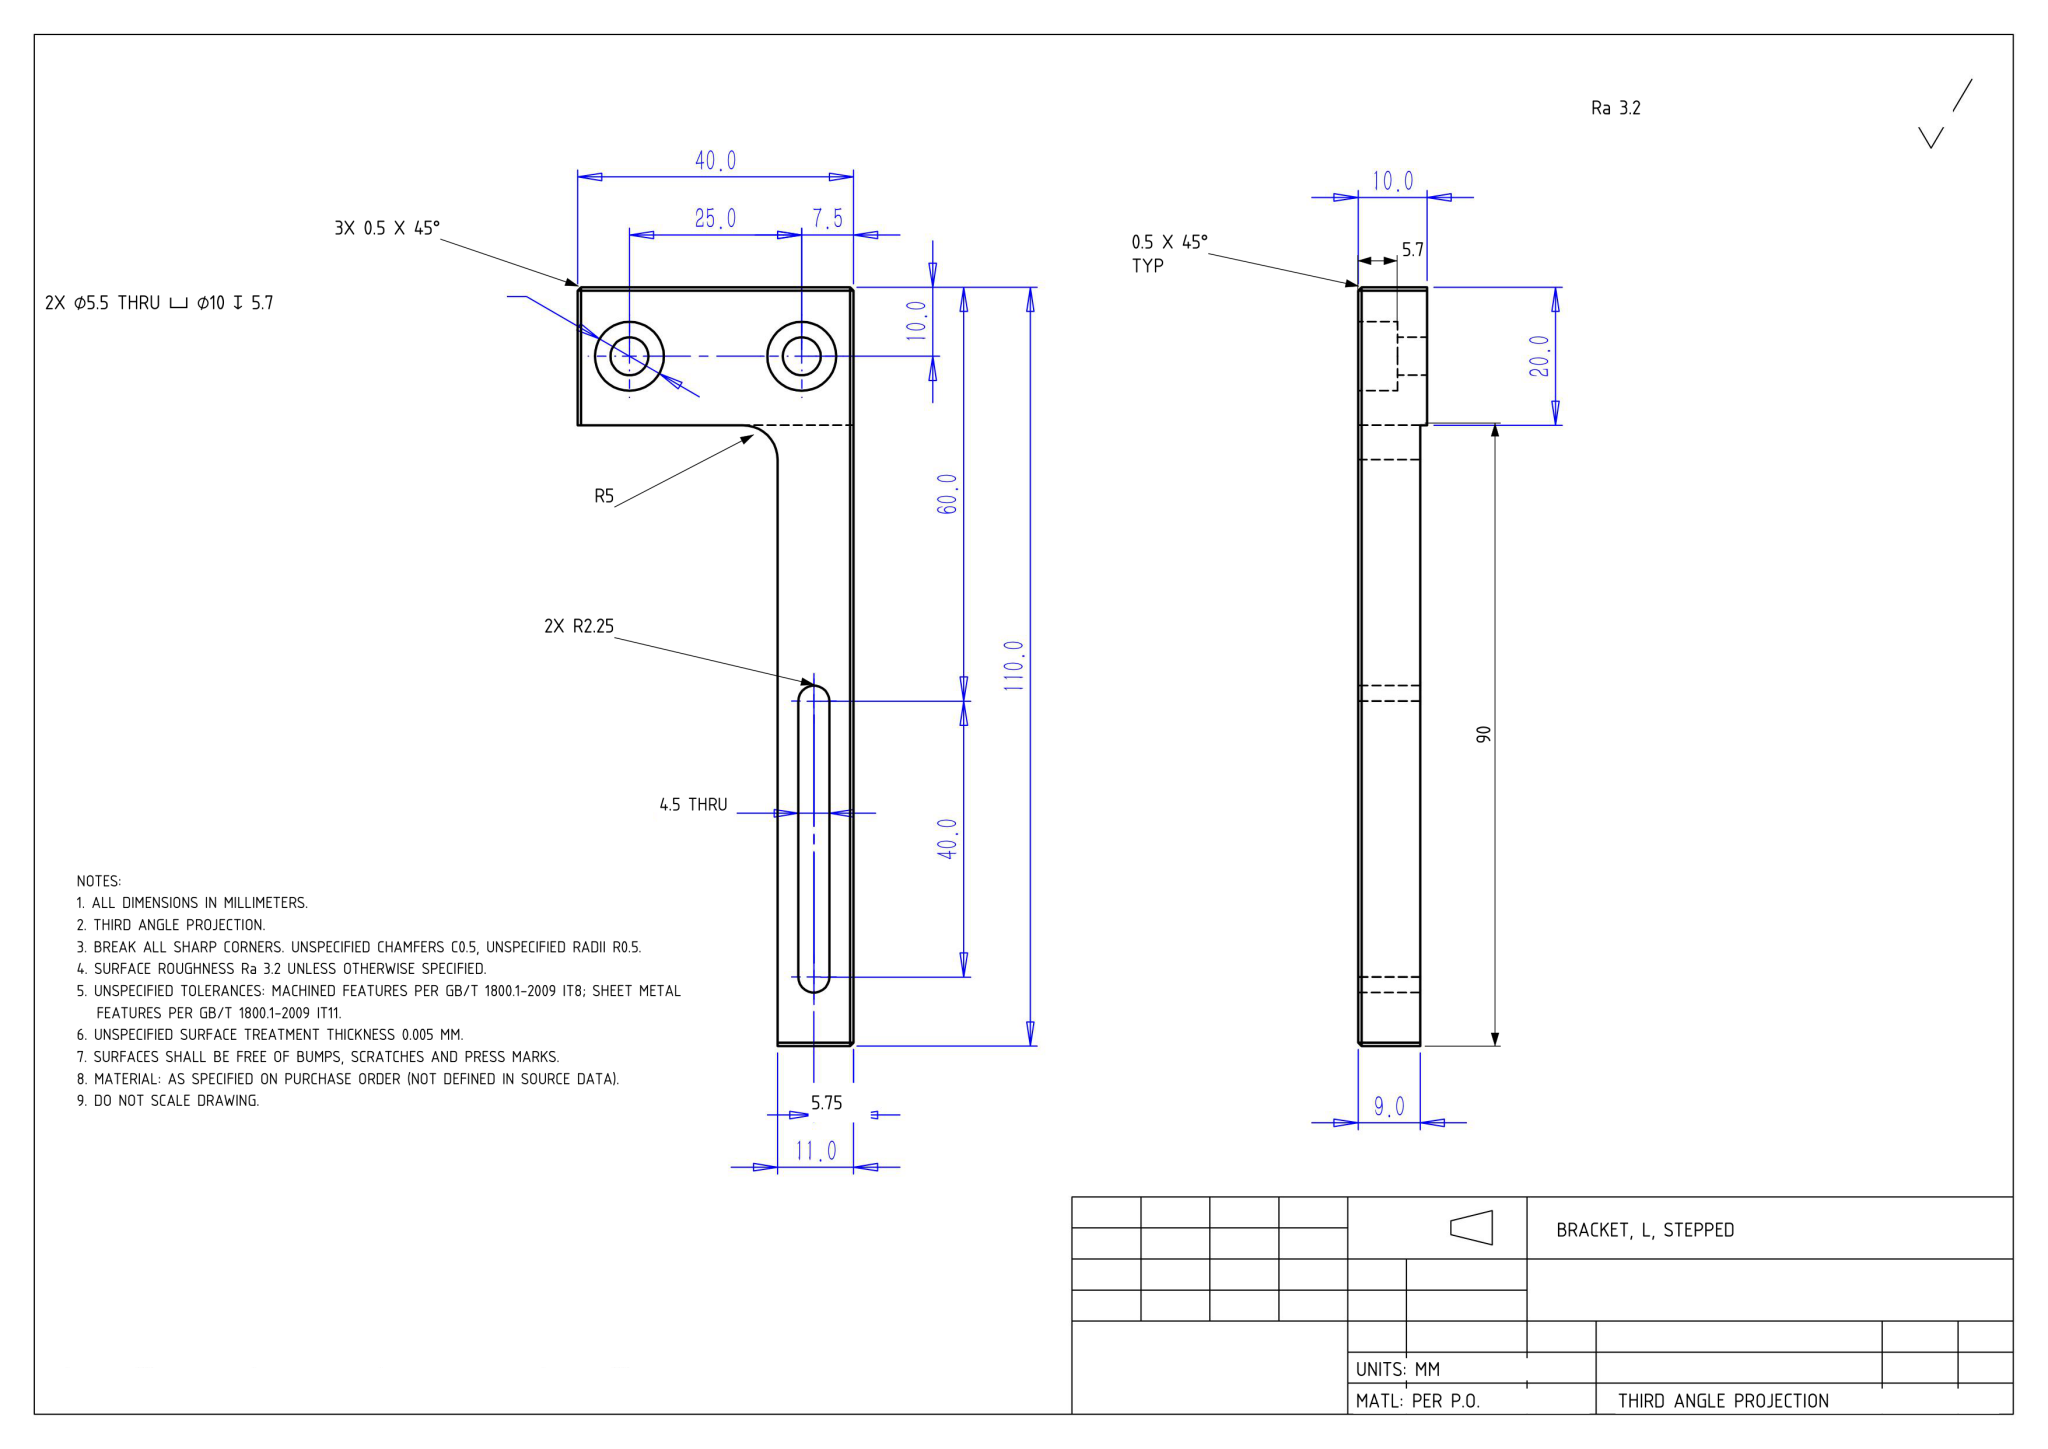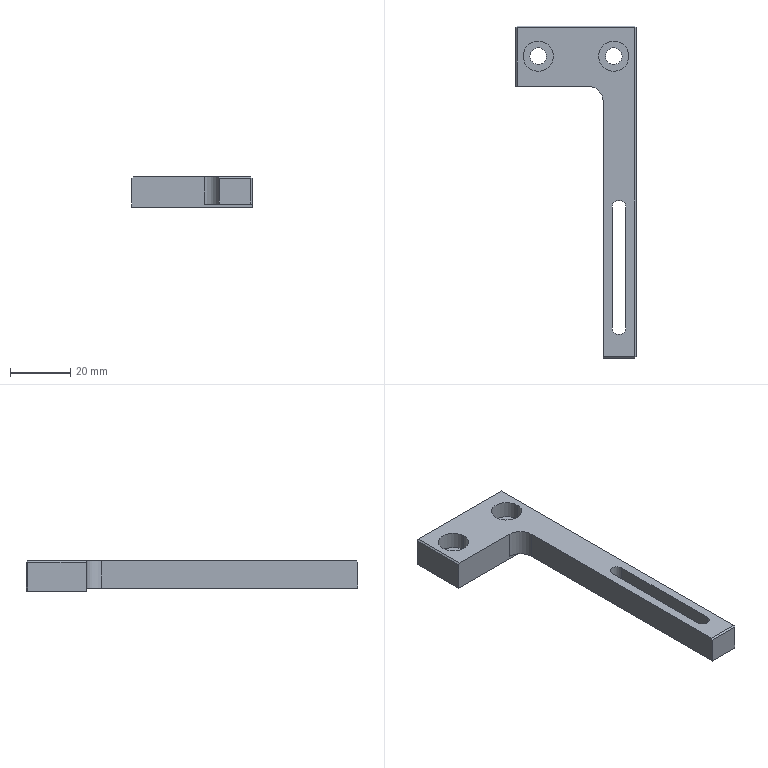Part | NX | mm | 1 solid | 34 faces | box 40 x 110 x 10 mm | volume 14069 mm3 | plane 23 | cylinder 11 | commonest cylinder face diameters 10 x5 5.5 x4 4.5 x2
STEP:
#1=COLOUR_RGB('',0.502,1.,1.);
#2=FILL_AREA_STYLE_COLOUR('',#1);
#3=FILL_AREA_STYLE('',(#2));
#4=SURFACE_STYLE_FILL_AREA(#3);
#5=SURFACE_SIDE_STYLE('',(#4));
#6=SURFACE_STYLE_USAGE(.BOTH.,#5);
#7=PRESENTATION_STYLE_ASSIGNMENT((#6));
#8=CARTESIAN_POINT('',(-17.5,45.,-0.7));
#9=VERTEX_POINT('',#8);
#10=CARTESIAN_POINT('',(-7.5,45.,-0.7));
#11=VERTEX_POINT('',#10);
#12=CARTESIAN_POINT('',(-12.5,45.,-0.7));
#13=DIRECTION('',(0.,0.,1.));
#14=DIRECTION('',(1.,0.,0.));
#15=AXIS2_PLACEMENT_3D('',#12,#13,#14);
#16=CIRCLE('',#15,5.);
#17=EDGE_CURVE('',#9,#11,#16,.T.);
#18=ORIENTED_EDGE('',*,*,#17,.F.);
#19=CARTESIAN_POINT('',(-17.5,45.,5.));
#20=VERTEX_POINT('',#19);
#21=CARTESIAN_POINT('',(-17.5,45.,5.));
#22=DIRECTION('',(0.,0.,1.));
#23=VECTOR('',#22,1000.);
#24=LINE('',#21,#23);
#25=EDGE_CURVE('',#9,#20,#24,.T.);
#26=ORIENTED_EDGE('',*,*,#25,.T.);
#27=CARTESIAN_POINT('',(-7.5,45.,5.));
#28=VERTEX_POINT('',#27);
#29=CARTESIAN_POINT('',(-12.5,45.,5.));
#30=DIRECTION('',(0.,0.,1.));
#31=DIRECTION('',(1.,0.,0.));
#32=AXIS2_PLACEMENT_3D('',#29,#30,#31);
#33=CIRCLE('',#32,5.);
#34=EDGE_CURVE('',#20,#28,#33,.T.);
#35=ORIENTED_EDGE('',*,*,#34,.T.);
#36=CARTESIAN_POINT('',(-7.5,45.,5.));
#37=DIRECTION('',(0.,0.,1.));
#38=VECTOR('',#37,1000.);
#39=LINE('',#36,#38);
#40=EDGE_CURVE('',#11,#28,#39,.T.);
#41=ORIENTED_EDGE('',*,*,#40,.F.);
#42=EDGE_LOOP('',(#18,#26,#35,#41));
#43=FACE_OUTER_BOUND('',#42,.T.);
#44=CARTESIAN_POINT('',(-12.5,45.,5.));
#45=DIRECTION('',(0.,0.,1.));
#46=DIRECTION('',(1.,0.,0.));
#47=AXIS2_PLACEMENT_3D('',#44,#45,#46);
#48=CYLINDRICAL_SURFACE('',#47,5.);
#49=ADVANCED_FACE('',(#43),#48,.F.);
#50=CARTESIAN_POINT('',(-15.25,45.,-5.));
#51=VERTEX_POINT('',#50);
#52=CARTESIAN_POINT('',(-9.75,45.,-5.));
#53=VERTEX_POINT('',#52);
#54=CARTESIAN_POINT('',(-12.5,45.,-5.));
#55=DIRECTION('',(0.,0.,1.));
#56=DIRECTION('',(1.,0.,0.));
#57=AXIS2_PLACEMENT_3D('',#54,#55,#56);
#58=CIRCLE('',#57,2.75);
#59=EDGE_CURVE('',#51,#53,#58,.T.);
#60=ORIENTED_EDGE('',*,*,#59,.F.);
#61=CARTESIAN_POINT('',(-15.25,45.,-0.7));
#62=VERTEX_POINT('',#61);
#63=CARTESIAN_POINT('',(-15.25,45.,5.));
#64=DIRECTION('',(0.,0.,1.));
#65=VECTOR('',#64,1000.);
#66=LINE('',#63,#65);
#67=EDGE_CURVE('',#51,#62,#66,.T.);
#68=ORIENTED_EDGE('',*,*,#67,.T.);
#69=CARTESIAN_POINT('',(-9.75,45.,-0.7));
#70=VERTEX_POINT('',#69);
#71=CARTESIAN_POINT('',(-12.5,45.,-0.7));
#72=DIRECTION('',(0.,0.,1.));
#73=DIRECTION('',(1.,0.,0.));
#74=AXIS2_PLACEMENT_3D('',#71,#72,#73);
#75=CIRCLE('',#74,2.75);
#76=EDGE_CURVE('',#62,#70,#75,.T.);
#77=ORIENTED_EDGE('',*,*,#76,.T.);
#78=CARTESIAN_POINT('',(-9.75,45.,5.));
#79=DIRECTION('',(0.,0.,1.));
#80=VECTOR('',#79,1000.);
#81=LINE('',#78,#80);
#82=EDGE_CURVE('',#53,#70,#81,.T.);
#83=ORIENTED_EDGE('',*,*,#82,.F.);
#84=EDGE_LOOP('',(#60,#68,#77,#83));
#85=FACE_OUTER_BOUND('',#84,.T.);
#86=CARTESIAN_POINT('',(-12.5,45.,5.));
#87=DIRECTION('',(0.,0.,1.));
#88=DIRECTION('',(1.,0.,0.));
#89=AXIS2_PLACEMENT_3D('',#86,#87,#88);
#90=CYLINDRICAL_SURFACE('',#89,2.75);
#91=ADVANCED_FACE('',(#85),#90,.F.);
#92=CARTESIAN_POINT('',(7.5,45.,-0.7));
#93=VERTEX_POINT('',#92);
#94=CARTESIAN_POINT('',(17.5,45.,-0.7));
#95=VERTEX_POINT('',#94);
#96=CARTESIAN_POINT('',(12.5,45.,-0.7));
#97=DIRECTION('',(0.,0.,1.));
#98=DIRECTION('',(1.,0.,0.));
#99=AXIS2_PLACEMENT_3D('',#96,#97,#98);
#100=CIRCLE('',#99,5.);
#101=EDGE_CURVE('',#93,#95,#100,.T.);
#102=ORIENTED_EDGE('',*,*,#101,.F.);
#103=CARTESIAN_POINT('',(7.5,45.,5.));
#104=VERTEX_POINT('',#103);
#105=CARTESIAN_POINT('',(7.5,45.,5.));
#106=DIRECTION('',(0.,0.,1.));
#107=VECTOR('',#106,1000.);
#108=LINE('',#105,#107);
#109=EDGE_CURVE('',#93,#104,#108,.T.);
#110=ORIENTED_EDGE('',*,*,#109,.T.);
#111=CARTESIAN_POINT('',(17.5,45.,5.));
#112=VERTEX_POINT('',#111);
#113=CARTESIAN_POINT('',(12.5,45.,5.));
#114=DIRECTION('',(0.,0.,1.));
#115=DIRECTION('',(1.,0.,0.));
#116=AXIS2_PLACEMENT_3D('',#113,#114,#115);
#117=CIRCLE('',#116,5.);
#118=EDGE_CURVE('',#104,#112,#117,.T.);
#119=ORIENTED_EDGE('',*,*,#118,.T.);
#120=CARTESIAN_POINT('',(17.5,45.,5.));
#121=DIRECTION('',(0.,0.,1.));
#122=VECTOR('',#121,1000.);
#123=LINE('',#120,#122);
#124=EDGE_CURVE('',#95,#112,#123,.T.);
#125=ORIENTED_EDGE('',*,*,#124,.F.);
#126=EDGE_LOOP('',(#102,#110,#119,#125));
#127=FACE_OUTER_BOUND('',#126,.T.);
#128=CARTESIAN_POINT('',(12.5,45.,5.));
#129=DIRECTION('',(0.,0.,1.));
#130=DIRECTION('',(1.,0.,0.));
#131=AXIS2_PLACEMENT_3D('',#128,#129,#130);
#132=CYLINDRICAL_SURFACE('',#131,5.);
#133=ADVANCED_FACE('',(#127),#132,.F.);
#134=CARTESIAN_POINT('',(9.75,45.,-5.));
#135=VERTEX_POINT('',#134);
#136=CARTESIAN_POINT('',(15.25,45.,-5.));
#137=VERTEX_POINT('',#136);
#138=CARTESIAN_POINT('',(12.5,45.,-5.));
#139=DIRECTION('',(0.,0.,1.));
#140=DIRECTION('',(1.,0.,0.));
#141=AXIS2_PLACEMENT_3D('',#138,#139,#140);
#142=CIRCLE('',#141,2.75);
#143=EDGE_CURVE('',#135,#137,#142,.T.);
#144=ORIENTED_EDGE('',*,*,#143,.F.);
#145=CARTESIAN_POINT('',(9.75,45.,-0.7));
#146=VERTEX_POINT('',#145);
#147=CARTESIAN_POINT('',(9.75,45.,5.));
#148=DIRECTION('',(0.,0.,1.));
#149=VECTOR('',#148,1000.);
#150=LINE('',#147,#149);
#151=EDGE_CURVE('',#135,#146,#150,.T.);
#152=ORIENTED_EDGE('',*,*,#151,.T.);
#153=CARTESIAN_POINT('',(15.25,45.,-0.7));
#154=VERTEX_POINT('',#153);
#155=CARTESIAN_POINT('',(12.5,45.,-0.7));
#156=DIRECTION('',(0.,0.,1.));
#157=DIRECTION('',(1.,0.,0.));
#158=AXIS2_PLACEMENT_3D('',#155,#156,#157);
#159=CIRCLE('',#158,2.75);
#160=EDGE_CURVE('',#146,#154,#159,.T.);
#161=ORIENTED_EDGE('',*,*,#160,.T.);
#162=CARTESIAN_POINT('',(15.25,45.,5.));
#163=DIRECTION('',(0.,0.,1.));
#164=VECTOR('',#163,1000.);
#165=LINE('',#162,#164);
#166=EDGE_CURVE('',#137,#154,#165,.T.);
#167=ORIENTED_EDGE('',*,*,#166,.F.);
#168=EDGE_LOOP('',(#144,#152,#161,#167));
#169=FACE_OUTER_BOUND('',#168,.T.);
#170=CARTESIAN_POINT('',(12.5,45.,5.));
#171=DIRECTION('',(0.,0.,1.));
#172=DIRECTION('',(1.,0.,0.));
#173=AXIS2_PLACEMENT_3D('',#170,#171,#172);
#174=CYLINDRICAL_SURFACE('',#173,2.75);
#175=ADVANCED_FACE('',(#169),#174,.F.);
#176=CARTESIAN_POINT('',(19.5,-55.,4.5));
#177=VERTEX_POINT('',#176);
#178=CARTESIAN_POINT('',(9.,-55.,4.5));
#179=VERTEX_POINT('',#178);
#180=CARTESIAN_POINT('',(-20.,-55.,4.5));
#181=DIRECTION('',(-1.,0.,0.));
#182=VECTOR('',#181,1000.);
#183=LINE('',#180,#182);
#184=EDGE_CURVE('',#177,#179,#183,.T.);
#185=ORIENTED_EDGE('',*,*,#184,.T.);
#186=CARTESIAN_POINT('',(9.,-55.,-4.));
#187=VERTEX_POINT('',#186);
#188=CARTESIAN_POINT('',(9.,-55.,5.));
#189=DIRECTION('',(0.,0.,-1.));
#190=VECTOR('',#189,1000.);
#191=LINE('',#188,#190);
#192=EDGE_CURVE('',#179,#187,#191,.T.);
#193=ORIENTED_EDGE('',*,*,#192,.T.);
#194=CARTESIAN_POINT('',(19.5,-55.,-4.));
#195=VERTEX_POINT('',#194);
#196=CARTESIAN_POINT('',(20.,-55.,-4.));
#197=DIRECTION('',(-1.,0.,0.));
#198=VECTOR('',#197,1000.);
#199=LINE('',#196,#198);
#200=EDGE_CURVE('',#195,#187,#199,.T.);
#201=ORIENTED_EDGE('',*,*,#200,.F.);
#202=CARTESIAN_POINT('',(19.5,-55.,5.));
#203=DIRECTION('',(0.,0.,1.));
#204=VECTOR('',#203,1000.);
#205=LINE('',#202,#204);
#206=EDGE_CURVE('',#195,#177,#205,.T.);
#207=ORIENTED_EDGE('',*,*,#206,.T.);
#208=EDGE_LOOP('',(#185,#193,#201,#207));
#209=FACE_OUTER_BOUND('',#208,.T.);
#210=CARTESIAN_POINT('',(-20.,-55.,5.));
#211=DIRECTION('',(0.,1.,0.));
#212=DIRECTION('',(0.,0.,1.));
#213=AXIS2_PLACEMENT_3D('',#210,#211,#212);
#214=PLANE('',#213);
#215=ADVANCED_FACE('',(#209),#214,.F.);
#216=ORIENTED_EDGE('',*,*,#206,.F.);
#217=CARTESIAN_POINT('',(20.,-54.5,-4.));
#218=VERTEX_POINT('',#217);
#219=CARTESIAN_POINT('',(20.,-54.5,-4.));
#220=DIRECTION('',(0.7071,0.7071,0.));
#221=VECTOR('',#220,1000.);
#222=LINE('',#219,#221);
#223=EDGE_CURVE('',#195,#218,#222,.T.);
#224=ORIENTED_EDGE('',*,*,#223,.T.);
#225=CARTESIAN_POINT('',(20.,-54.5,4.5));
#226=VERTEX_POINT('',#225);
#227=CARTESIAN_POINT('',(20.,-54.5,5.));
#228=DIRECTION('',(0.,0.,-1.));
#229=VECTOR('',#228,1000.);
#230=LINE('',#227,#229);
#231=EDGE_CURVE('',#226,#218,#230,.T.);
#232=ORIENTED_EDGE('',*,*,#231,.F.);
#233=CARTESIAN_POINT('',(19.75,-54.75,4.5));
#234=DIRECTION('',(0.7071,0.7071,0.));
#235=VECTOR('',#234,1000.);
#236=LINE('',#233,#235);
#237=EDGE_CURVE('',#177,#226,#236,.T.);
#238=ORIENTED_EDGE('',*,*,#237,.F.);
#239=EDGE_LOOP('',(#216,#224,#232,#238));
#240=FACE_OUTER_BOUND('',#239,.T.);
#241=CARTESIAN_POINT('',(20.,-54.5,5.));
#242=DIRECTION('',(-0.7071,0.7071,0.));
#243=DIRECTION('',(0.,0.,-1.));
#244=AXIS2_PLACEMENT_3D('',#241,#242,#243);
#245=PLANE('',#244);
#246=ADVANCED_FACE('',(#240),#245,.F.);
#247=CARTESIAN_POINT('',(20.,35.,-4.));
#248=VERTEX_POINT('',#247);
#249=CARTESIAN_POINT('',(20.,35.,-4.));
#250=DIRECTION('',(-0.,-1.,0.));
#251=VECTOR('',#250,1000.);
#252=LINE('',#249,#251);
#253=EDGE_CURVE('',#248,#218,#252,.T.);
#254=ORIENTED_EDGE('',*,*,#253,.F.);
#255=CARTESIAN_POINT('',(20.,35.,-5.));
#256=VERTEX_POINT('',#255);
#257=CARTESIAN_POINT('',(20.,35.,-4.));
#258=DIRECTION('',(0.,0.,-1.));
#259=VECTOR('',#258,1000.);
#260=LINE('',#257,#259);
#261=EDGE_CURVE('',#248,#256,#260,.T.);
#262=ORIENTED_EDGE('',*,*,#261,.T.);
#263=CARTESIAN_POINT('',(20.,54.5,-5.));
#264=VERTEX_POINT('',#263);
#265=CARTESIAN_POINT('',(20.,-55.,-5.));
#266=DIRECTION('',(0.,1.,0.));
#267=VECTOR('',#266,1000.);
#268=LINE('',#265,#267);
#269=EDGE_CURVE('',#256,#264,#268,.T.);
#270=ORIENTED_EDGE('',*,*,#269,.T.);
#271=CARTESIAN_POINT('',(20.,54.5,4.5));
#272=VERTEX_POINT('',#271);
#273=CARTESIAN_POINT('',(20.,54.5,5.));
#274=DIRECTION('',(0.,0.,1.));
#275=VECTOR('',#274,1000.);
#276=LINE('',#273,#275);
#277=EDGE_CURVE('',#264,#272,#276,.T.);
#278=ORIENTED_EDGE('',*,*,#277,.T.);
#279=CARTESIAN_POINT('',(20.,-55.,4.5));
#280=DIRECTION('',(0.,-1.,0.));
#281=VECTOR('',#280,1000.);
#282=LINE('',#279,#281);
#283=EDGE_CURVE('',#272,#226,#282,.T.);
#284=ORIENTED_EDGE('',*,*,#283,.T.);
#285=ORIENTED_EDGE('',*,*,#231,.T.);
#286=EDGE_LOOP('',(#254,#262,#270,#278,#284,#285));
#287=FACE_OUTER_BOUND('',#286,.T.);
#288=CARTESIAN_POINT('',(20.,-55.,5.));
#289=DIRECTION('',(-1.,0.,0.));
#290=DIRECTION('',(0.,0.,1.));
#291=AXIS2_PLACEMENT_3D('',#288,#289,#290);
#292=PLANE('',#291);
#293=ADVANCED_FACE('',(#287),#292,.F.);
#294=CARTESIAN_POINT('',(-19.5,55.,4.5));
#295=VERTEX_POINT('',#294);
#296=CARTESIAN_POINT('',(19.5,55.,4.5));
#297=VERTEX_POINT('',#296);
#298=CARTESIAN_POINT('',(-20.,55.,4.5));
#299=DIRECTION('',(1.,0.,0.));
#300=VECTOR('',#299,1000.);
#301=LINE('',#298,#300);
#302=EDGE_CURVE('',#295,#297,#301,.T.);
#303=ORIENTED_EDGE('',*,*,#302,.T.);
#304=CARTESIAN_POINT('',(19.5,55.,-5.));
#305=VERTEX_POINT('',#304);
#306=CARTESIAN_POINT('',(19.5,55.,5.));
#307=DIRECTION('',(0.,0.,-1.));
#308=VECTOR('',#307,1000.);
#309=LINE('',#306,#308);
#310=EDGE_CURVE('',#297,#305,#309,.T.);
#311=ORIENTED_EDGE('',*,*,#310,.T.);
#312=CARTESIAN_POINT('',(-19.5,55.,-5.));
#313=VERTEX_POINT('',#312);
#314=CARTESIAN_POINT('',(-20.,55.,-5.));
#315=DIRECTION('',(-1.,0.,0.));
#316=VECTOR('',#315,1000.);
#317=LINE('',#314,#316);
#318=EDGE_CURVE('',#305,#313,#317,.T.);
#319=ORIENTED_EDGE('',*,*,#318,.T.);
#320=CARTESIAN_POINT('',(-19.5,55.,5.));
#321=DIRECTION('',(0.,0.,1.));
#322=VECTOR('',#321,1000.);
#323=LINE('',#320,#322);
#324=EDGE_CURVE('',#313,#295,#323,.T.);
#325=ORIENTED_EDGE('',*,*,#324,.T.);
#326=EDGE_LOOP('',(#303,#311,#319,#325));
#327=FACE_OUTER_BOUND('',#326,.T.);
#328=CARTESIAN_POINT('',(-20.,55.,5.));
#329=DIRECTION('',(0.,-1.,0.));
#330=DIRECTION('',(0.,0.,-1.));
#331=AXIS2_PLACEMENT_3D('',#328,#329,#330);
#332=PLANE('',#331);
#333=ADVANCED_FACE('',(#327),#332,.F.);
#334=CARTESIAN_POINT('',(-20.,35.,4.5));
#335=VERTEX_POINT('',#334);
#336=CARTESIAN_POINT('',(-20.,35.,-5.));
#337=VERTEX_POINT('',#336);
#338=CARTESIAN_POINT('',(-20.,35.,-4.));
#339=DIRECTION('',(0.,0.,-1.));
#340=VECTOR('',#339,1000.);
#341=LINE('',#338,#340);
#342=EDGE_CURVE('',#335,#337,#341,.T.);
#343=ORIENTED_EDGE('',*,*,#342,.F.);
#344=CARTESIAN_POINT('',(-20.,54.5,4.5));
#345=VERTEX_POINT('',#344);
#346=CARTESIAN_POINT('',(-20.,-55.,4.5));
#347=DIRECTION('',(0.,1.,0.));
#348=VECTOR('',#347,1000.);
#349=LINE('',#346,#348);
#350=EDGE_CURVE('',#335,#345,#349,.T.);
#351=ORIENTED_EDGE('',*,*,#350,.T.);
#352=CARTESIAN_POINT('',(-20.,54.5,-5.));
#353=VERTEX_POINT('',#352);
#354=CARTESIAN_POINT('',(-20.,54.5,5.));
#355=DIRECTION('',(0.,0.,-1.));
#356=VECTOR('',#355,1000.);
#357=LINE('',#354,#356);
#358=EDGE_CURVE('',#345,#353,#357,.T.);
#359=ORIENTED_EDGE('',*,*,#358,.T.);
#360=CARTESIAN_POINT('',(-20.,-55.,-5.));
#361=DIRECTION('',(0.,-1.,0.));
#362=VECTOR('',#361,1000.);
#363=LINE('',#360,#362);
#364=EDGE_CURVE('',#353,#337,#363,.T.);
#365=ORIENTED_EDGE('',*,*,#364,.T.);
#366=EDGE_LOOP('',(#343,#351,#359,#365));
#367=FACE_OUTER_BOUND('',#366,.T.);
#368=CARTESIAN_POINT('',(-20.,-55.,5.));
#369=DIRECTION('',(1.,0.,0.));
#370=DIRECTION('',(0.,0.,-1.));
#371=AXIS2_PLACEMENT_3D('',#368,#369,#370);
#372=PLANE('',#371);
#373=ADVANCED_FACE('',(#367),#372,.F.);
#374=CARTESIAN_POINT('',(12.,-5.,5.));
#375=VERTEX_POINT('',#374);
#376=CARTESIAN_POINT('',(12.,-45.,5.));
#377=VERTEX_POINT('',#376);
#378=CARTESIAN_POINT('',(12.,-5.,5.));
#379=DIRECTION('',(0.,-1.,0.));
#380=VECTOR('',#379,1000.);
#381=LINE('',#378,#380);
#382=EDGE_CURVE('',#375,#377,#381,.T.);
#383=ORIENTED_EDGE('',*,*,#382,.F.);
#384=CARTESIAN_POINT('',(16.5,-5.,5.));
#385=VERTEX_POINT('',#384);
#386=CARTESIAN_POINT('',(14.25,-5.,5.));
#387=DIRECTION('',(0.,0.,1.));
#388=DIRECTION('',(1.,0.,0.));
#389=AXIS2_PLACEMENT_3D('',#386,#387,#388);
#390=CIRCLE('',#389,2.25);
#391=EDGE_CURVE('',#385,#375,#390,.T.);
#392=ORIENTED_EDGE('',*,*,#391,.F.);
#393=CARTESIAN_POINT('',(16.5,-45.,5.));
#394=VERTEX_POINT('',#393);
#395=CARTESIAN_POINT('',(16.5,-5.,5.));
#396=DIRECTION('',(-0.,1.,0.));
#397=VECTOR('',#396,1000.);
#398=LINE('',#395,#397);
#399=EDGE_CURVE('',#394,#385,#398,.T.);
#400=ORIENTED_EDGE('',*,*,#399,.F.);
#401=CARTESIAN_POINT('',(14.25,-45.,5.));
#402=DIRECTION('',(0.,0.,1.));
#403=DIRECTION('',(1.,0.,0.));
#404=AXIS2_PLACEMENT_3D('',#401,#402,#403);
#405=CIRCLE('',#404,2.25);
#406=EDGE_CURVE('',#377,#394,#405,.T.);
#407=ORIENTED_EDGE('',*,*,#406,.F.);
#408=EDGE_LOOP('',(#383,#392,#400,#407));
#409=FACE_BOUND('',#408,.T.);
#410=CARTESIAN_POINT('',(-12.5,45.,5.));
#411=DIRECTION('',(0.,0.,1.));
#412=DIRECTION('',(1.,0.,0.));
#413=AXIS2_PLACEMENT_3D('',#410,#411,#412);
#414=CIRCLE('',#413,5.);
#415=EDGE_CURVE('',#28,#20,#414,.T.);
#416=ORIENTED_EDGE('',*,*,#415,.F.);
#417=ORIENTED_EDGE('',*,*,#34,.F.);
#418=EDGE_LOOP('',(#416,#417));
#419=FACE_BOUND('',#418,.T.);
#420=CARTESIAN_POINT('',(12.5,45.,5.));
#421=DIRECTION('',(0.,0.,1.));
#422=DIRECTION('',(1.,0.,0.));
#423=AXIS2_PLACEMENT_3D('',#420,#421,#422);
#424=CIRCLE('',#423,5.);
#425=EDGE_CURVE('',#112,#104,#424,.T.);
#426=ORIENTED_EDGE('',*,*,#425,.F.);
#427=ORIENTED_EDGE('',*,*,#118,.F.);
#428=EDGE_LOOP('',(#426,#427));
#429=FACE_BOUND('',#428,.T.);
#430=CARTESIAN_POINT('',(-19.5,35.,5.));
#431=VERTEX_POINT('',#430);
#432=CARTESIAN_POINT('',(4.,35.,5.));
#433=VERTEX_POINT('',#432);
#434=CARTESIAN_POINT('',(9.,35.,5.));
#435=DIRECTION('',(1.,0.,0.));
#436=VECTOR('',#435,1000.);
#437=LINE('',#434,#436);
#438=EDGE_CURVE('',#431,#433,#437,.T.);
#439=ORIENTED_EDGE('',*,*,#438,.T.);
#440=CARTESIAN_POINT('',(9.,30.,5.));
#441=VERTEX_POINT('',#440);
#442=CARTESIAN_POINT('',(4.,30.,5.));
#443=DIRECTION('',(0.,0.,-1.));
#444=DIRECTION('',(-1.,0.,0.));
#445=AXIS2_PLACEMENT_3D('',#442,#443,#444);
#446=CIRCLE('',#445,5.);
#447=EDGE_CURVE('',#433,#441,#446,.T.);
#448=ORIENTED_EDGE('',*,*,#447,.T.);
#449=CARTESIAN_POINT('',(9.,-54.5,5.));
#450=VERTEX_POINT('',#449);
#451=CARTESIAN_POINT('',(9.,35.,5.));
#452=DIRECTION('',(-0.,-1.,0.));
#453=VECTOR('',#452,1000.);
#454=LINE('',#451,#453);
#455=EDGE_CURVE('',#441,#450,#454,.T.);
#456=ORIENTED_EDGE('',*,*,#455,.T.);
#457=CARTESIAN_POINT('',(19.5,-54.5,5.));
#458=VERTEX_POINT('',#457);
#459=CARTESIAN_POINT('',(0.,-54.5,5.));
#460=DIRECTION('',(1.,0.,0.));
#461=VECTOR('',#460,1000.);
#462=LINE('',#459,#461);
#463=EDGE_CURVE('',#450,#458,#462,.T.);
#464=ORIENTED_EDGE('',*,*,#463,.T.);
#465=CARTESIAN_POINT('',(19.5,54.5,5.));
#466=VERTEX_POINT('',#465);
#467=CARTESIAN_POINT('',(19.5,0.,5.));
#468=DIRECTION('',(0.,1.,0.));
#469=VECTOR('',#468,1000.);
#470=LINE('',#467,#469);
#471=EDGE_CURVE('',#458,#466,#470,.T.);
#472=ORIENTED_EDGE('',*,*,#471,.T.);
#473=CARTESIAN_POINT('',(-19.5,54.5,5.));
#474=VERTEX_POINT('',#473);
#475=CARTESIAN_POINT('',(0.,54.5,5.));
#476=DIRECTION('',(-1.,0.,0.));
#477=VECTOR('',#476,1000.);
#478=LINE('',#475,#477);
#479=EDGE_CURVE('',#466,#474,#478,.T.);
#480=ORIENTED_EDGE('',*,*,#479,.T.);
#481=CARTESIAN_POINT('',(-19.5,0.,5.));
#482=DIRECTION('',(0.,-1.,0.));
#483=VECTOR('',#482,1000.);
#484=LINE('',#481,#483);
#485=EDGE_CURVE('',#474,#431,#484,.T.);
#486=ORIENTED_EDGE('',*,*,#485,.T.);
#487=EDGE_LOOP('',(#439,#448,#456,#464,#472,#480,#486));
#488=FACE_OUTER_BOUND('',#487,.T.);
#489=CARTESIAN_POINT('',(0.,0.,5.));
#490=DIRECTION('',(0.,0.,-1.));
#491=DIRECTION('',(-1.,0.,0.));
#492=AXIS2_PLACEMENT_3D('',#489,#490,#491);
#493=PLANE('',#492);
#494=ADVANCED_FACE('',(#409,#419,#429,#488),#493,.F.);
#495=CARTESIAN_POINT('',(20.,35.,-5.));
#496=DIRECTION('',(1.,-0.,0.));
#497=VECTOR('',#496,1000.);
#498=LINE('',#495,#497);
#499=EDGE_CURVE('',#337,#256,#498,.T.);
#500=ORIENTED_EDGE('',*,*,#499,.F.);
#501=ORIENTED_EDGE('',*,*,#364,.F.);
#502=CARTESIAN_POINT('',(-37.25,37.25,-5.));
#503=DIRECTION('',(0.7071,0.7071,0.));
#504=VECTOR('',#503,1000.);
#505=LINE('',#502,#504);
#506=EDGE_CURVE('',#353,#313,#505,.T.);
#507=ORIENTED_EDGE('',*,*,#506,.T.);
#508=ORIENTED_EDGE('',*,*,#318,.F.);
#509=CARTESIAN_POINT('',(37.25,37.25,-5.));
#510=DIRECTION('',(0.7071,-0.7071,0.));
#511=VECTOR('',#510,1000.);
#512=LINE('',#509,#511);
#513=EDGE_CURVE('',#305,#264,#512,.T.);
#514=ORIENTED_EDGE('',*,*,#513,.T.);
#515=ORIENTED_EDGE('',*,*,#269,.F.);
#516=EDGE_LOOP('',(#500,#501,#507,#508,#514,#515));
#517=FACE_OUTER_BOUND('',#516,.T.);
#518=CARTESIAN_POINT('',(-12.5,45.,-5.));
#519=DIRECTION('',(0.,0.,1.));
#520=DIRECTION('',(1.,0.,0.));
#521=AXIS2_PLACEMENT_3D('',#518,#519,#520);
#522=CIRCLE('',#521,2.75);
#523=EDGE_CURVE('',#53,#51,#522,.T.);
#524=ORIENTED_EDGE('',*,*,#523,.T.);
#525=ORIENTED_EDGE('',*,*,#59,.T.);
#526=EDGE_LOOP('',(#524,#525));
#527=FACE_BOUND('',#526,.T.);
#528=CARTESIAN_POINT('',(12.5,45.,-5.));
#529=DIRECTION('',(0.,0.,1.));
#530=DIRECTION('',(1.,0.,0.));
#531=AXIS2_PLACEMENT_3D('',#528,#529,#530);
#532=CIRCLE('',#531,2.75);
#533=EDGE_CURVE('',#137,#135,#532,.T.);
#534=ORIENTED_EDGE('',*,*,#533,.T.);
#535=ORIENTED_EDGE('',*,*,#143,.T.);
#536=EDGE_LOOP('',(#534,#535));
#537=FACE_BOUND('',#536,.T.);
#538=CARTESIAN_POINT('',(0.,0.,-5.));
#539=DIRECTION('',(0.,0.,-1.));
#540=DIRECTION('',(-1.,0.,0.));
#541=AXIS2_PLACEMENT_3D('',#538,#539,#540);
#542=PLANE('',#541);
#543=ADVANCED_FACE('',(#517,#527,#537),#542,.T.);
#544=ORIENTED_EDGE('',*,*,#506,.F.);
#545=ORIENTED_EDGE('',*,*,#358,.F.);
#546=CARTESIAN_POINT('',(-19.75,54.75,4.5));
#547=DIRECTION('',(-0.7071,-0.7071,0.));
#548=VECTOR('',#547,1000.);
#549=LINE('',#546,#548);
#550=EDGE_CURVE('',#295,#345,#549,.T.);
#551=ORIENTED_EDGE('',*,*,#550,.F.);
#552=ORIENTED_EDGE('',*,*,#324,.F.);
#553=EDGE_LOOP('',(#544,#545,#551,#552));
#554=FACE_OUTER_BOUND('',#553,.T.);
#555=CARTESIAN_POINT('',(-20.,54.5,5.));
#556=DIRECTION('',(0.7071,-0.7071,0.));
#557=DIRECTION('',(0.,0.,-1.));
#558=AXIS2_PLACEMENT_3D('',#555,#556,#557);
#559=PLANE('',#558);
#560=ADVANCED_FACE('',(#554),#559,.F.);
#561=CARTESIAN_POINT('',(19.5,54.5,5.));
#562=DIRECTION('',(-0.,-0.7071,0.7071));
#563=VECTOR('',#562,1000.);
#564=LINE('',#561,#563);
#565=EDGE_CURVE('',#297,#466,#564,.T.);
#566=ORIENTED_EDGE('',*,*,#565,.F.);
#567=ORIENTED_EDGE('',*,*,#302,.F.);
#568=CARTESIAN_POINT('',(-19.5,54.5,5.));
#569=DIRECTION('',(0.,0.7071,-0.7071));
#570=VECTOR('',#569,1000.);
#571=LINE('',#568,#570);
#572=EDGE_CURVE('',#474,#295,#571,.T.);
#573=ORIENTED_EDGE('',*,*,#572,.F.);
#574=ORIENTED_EDGE('',*,*,#479,.F.);
#575=EDGE_LOOP('',(#566,#567,#573,#574));
#576=FACE_OUTER_BOUND('',#575,.T.);
#577=CARTESIAN_POINT('',(0.,54.5,5.));
#578=DIRECTION('',(0.,-0.7071,-0.7071));
#579=DIRECTION('',(-1.,0.,0.));
#580=AXIS2_PLACEMENT_3D('',#577,#578,#579);
#581=PLANE('',#580);
#582=ADVANCED_FACE('',(#576),#581,.F.);
#583=ORIENTED_EDGE('',*,*,#513,.F.);
#584=ORIENTED_EDGE('',*,*,#310,.F.);
#585=CARTESIAN_POINT('',(19.75,54.75,4.5));
#586=DIRECTION('',(-0.7071,0.7071,0.));
#587=VECTOR('',#586,1000.);
#588=LINE('',#585,#587);
#589=EDGE_CURVE('',#272,#297,#588,.T.);
#590=ORIENTED_EDGE('',*,*,#589,.F.);
#591=ORIENTED_EDGE('',*,*,#277,.F.);
#592=EDGE_LOOP('',(#583,#584,#590,#591));
#593=FACE_OUTER_BOUND('',#592,.T.);
#594=CARTESIAN_POINT('',(19.5,55.,5.));
#595=DIRECTION('',(-0.7071,-0.7071,0.));
#596=DIRECTION('',(0.,0.,-1.));
#597=AXIS2_PLACEMENT_3D('',#594,#595,#596);
#598=PLANE('',#597);
#599=ADVANCED_FACE('',(#593),#598,.F.);
#600=ORIENTED_EDGE('',*,*,#572,.T.);
#601=ORIENTED_EDGE('',*,*,#550,.T.);
#602=CARTESIAN_POINT('',(-19.5,54.5,5.));
#603=DIRECTION('',(-0.7071,0.,-0.7071));
#604=VECTOR('',#603,1000.);
#605=LINE('',#602,#604);
#606=EDGE_CURVE('',#474,#345,#605,.T.);
#607=ORIENTED_EDGE('',*,*,#606,.F.);
#608=EDGE_LOOP('',(#600,#601,#607));
#609=FACE_OUTER_BOUND('',#608,.T.);
#610=CARTESIAN_POINT('',(-19.5,54.5,5.));
#611=DIRECTION('',(-0.5774,0.5774,0.5774));
#612=DIRECTION('',(0.7071,0.,0.7071));
#613=AXIS2_PLACEMENT_3D('',#610,#611,#612);
#614=PLANE('',#613);
#615=ADVANCED_FACE('',(#609),#614,.T.);
#616=ORIENTED_EDGE('',*,*,#589,.T.);
#617=ORIENTED_EDGE('',*,*,#565,.T.);
#618=CARTESIAN_POINT('',(19.5,54.5,5.));
#619=DIRECTION('',(-0.7071,0.,0.7071));
#620=VECTOR('',#619,1000.);
#621=LINE('',#618,#620);
#622=EDGE_CURVE('',#272,#466,#621,.T.);
#623=ORIENTED_EDGE('',*,*,#622,.F.);
#624=EDGE_LOOP('',(#616,#617,#623));
#625=FACE_OUTER_BOUND('',#624,.T.);
#626=CARTESIAN_POINT('',(19.5,54.5,5.));
#627=DIRECTION('',(0.5774,0.5774,0.5774));
#628=DIRECTION('',(0.7071,0.,-0.7071));
#629=AXIS2_PLACEMENT_3D('',#626,#627,#628);
#630=PLANE('',#629);
#631=ADVANCED_FACE('',(#625),#630,.T.);
#632=CARTESIAN_POINT('',(-19.5,35.,5.));
#633=DIRECTION('',(-0.7071,0.,-0.7071));
#634=VECTOR('',#633,1000.);
#635=LINE('',#632,#634);
#636=EDGE_CURVE('',#431,#335,#635,.T.);
#637=ORIENTED_EDGE('',*,*,#636,.F.);
#638=ORIENTED_EDGE('',*,*,#485,.F.);
#639=ORIENTED_EDGE('',*,*,#606,.T.);
#640=ORIENTED_EDGE('',*,*,#350,.F.);
#641=EDGE_LOOP('',(#637,#638,#639,#640));
#642=FACE_OUTER_BOUND('',#641,.T.);
#643=CARTESIAN_POINT('',(-19.5,0.,5.));
#644=DIRECTION('',(0.7071,0.,-0.7071));
#645=DIRECTION('',(0.,-1.,0.));
#646=AXIS2_PLACEMENT_3D('',#643,#644,#645);
#647=PLANE('',#646);
#648=ADVANCED_FACE('',(#642),#647,.F.);
#649=ORIENTED_EDGE('',*,*,#622,.T.);
#650=ORIENTED_EDGE('',*,*,#471,.F.);
#651=CARTESIAN_POINT('',(19.5,-54.5,5.));
#652=DIRECTION('',(-0.7071,0.,0.7071));
#653=VECTOR('',#652,1000.);
#654=LINE('',#651,#653);
#655=EDGE_CURVE('',#226,#458,#654,.T.);
#656=ORIENTED_EDGE('',*,*,#655,.F.);
#657=ORIENTED_EDGE('',*,*,#283,.F.);
#658=EDGE_LOOP('',(#649,#650,#656,#657));
#659=FACE_OUTER_BOUND('',#658,.T.);
#660=CARTESIAN_POINT('',(19.5,0.,5.));
#661=DIRECTION('',(-0.7071,0.,-0.7071));
#662=DIRECTION('',(0.,1.,0.));
#663=AXIS2_PLACEMENT_3D('',#660,#661,#662);
#664=PLANE('',#663);
#665=ADVANCED_FACE('',(#659),#664,.F.);
#666=ORIENTED_EDGE('',*,*,#237,.T.);
#667=ORIENTED_EDGE('',*,*,#655,.T.);
#668=CARTESIAN_POINT('',(19.5,-54.5,5.));
#669=DIRECTION('',(-0.,0.7071,0.7071));
#670=VECTOR('',#669,1000.);
#671=LINE('',#668,#670);
#672=EDGE_CURVE('',#177,#458,#671,.T.);
#673=ORIENTED_EDGE('',*,*,#672,.F.);
#674=EDGE_LOOP('',(#666,#667,#673));
#675=FACE_OUTER_BOUND('',#674,.T.);
#676=CARTESIAN_POINT('',(19.5,-54.5,5.));
#677=DIRECTION('',(0.5774,-0.5774,0.5774));
#678=DIRECTION('',(0.7071,0.,-0.7071));
#679=AXIS2_PLACEMENT_3D('',#676,#677,#678);
#680=PLANE('',#679);
#681=ADVANCED_FACE('',(#675),#680,.T.);
#682=CARTESIAN_POINT('',(9.,-54.5,5.));
#683=DIRECTION('',(0.,0.7071,0.7071));
#684=VECTOR('',#683,1000.);
#685=LINE('',#682,#684);
#686=EDGE_CURVE('',#179,#450,#685,.T.);
#687=ORIENTED_EDGE('',*,*,#686,.F.);
#688=ORIENTED_EDGE('',*,*,#184,.F.);
#689=ORIENTED_EDGE('',*,*,#672,.T.);
#690=ORIENTED_EDGE('',*,*,#463,.F.);
#691=EDGE_LOOP('',(#687,#688,#689,#690));
#692=FACE_OUTER_BOUND('',#691,.T.);
#693=CARTESIAN_POINT('',(0.,-54.5,5.));
#694=DIRECTION('',(0.,0.7071,-0.7071));
#695=DIRECTION('',(1.,0.,0.));
#696=AXIS2_PLACEMENT_3D('',#693,#694,#695);
#697=PLANE('',#696);
#698=ADVANCED_FACE('',(#692),#697,.F.);
#699=ORIENTED_EDGE('',*,*,#151,.F.);
#700=ORIENTED_EDGE('',*,*,#533,.F.);
#701=ORIENTED_EDGE('',*,*,#166,.T.);
#702=CARTESIAN_POINT('',(12.5,45.,-0.7));
#703=DIRECTION('',(0.,0.,1.));
#704=DIRECTION('',(1.,0.,0.));
#705=AXIS2_PLACEMENT_3D('',#702,#703,#704);
#706=CIRCLE('',#705,2.75);
#707=EDGE_CURVE('',#154,#146,#706,.T.);
#708=ORIENTED_EDGE('',*,*,#707,.T.);
#709=EDGE_LOOP('',(#699,#700,#701,#708));
#710=FACE_OUTER_BOUND('',#709,.T.);
#711=CARTESIAN_POINT('',(12.5,45.,5.));
#712=DIRECTION('',(0.,0.,1.));
#713=DIRECTION('',(1.,0.,0.));
#714=AXIS2_PLACEMENT_3D('',#711,#712,#713);
#715=CYLINDRICAL_SURFACE('',#714,2.75);
#716=ADVANCED_FACE('',(#710),#715,.F.);
#717=ORIENTED_EDGE('',*,*,#707,.F.);
#718=ORIENTED_EDGE('',*,*,#160,.F.);
#719=EDGE_LOOP('',(#717,#718));
#720=FACE_BOUND('',#719,.T.);
#721=CARTESIAN_POINT('',(12.5,45.,-0.7));
#722=DIRECTION('',(0.,0.,1.));
#723=DIRECTION('',(1.,0.,0.));
#724=AXIS2_PLACEMENT_3D('',#721,#722,#723);
#725=CIRCLE('',#724,5.);
#726=EDGE_CURVE('',#95,#93,#725,.T.);
#727=ORIENTED_EDGE('',*,*,#726,.T.);
#728=ORIENTED_EDGE('',*,*,#101,.T.);
#729=EDGE_LOOP('',(#727,#728));
#730=FACE_OUTER_BOUND('',#729,.T.);
#731=CARTESIAN_POINT('',(15.25,45.,-0.7));
#732=DIRECTION('',(0.,0.,-1.));
#733=DIRECTION('',(-1.,0.,0.));
#734=AXIS2_PLACEMENT_3D('',#731,#732,#733);
#735=PLANE('',#734);
#736=ADVANCED_FACE('',(#720,#730),#735,.F.);
#737=ORIENTED_EDGE('',*,*,#109,.F.);
#738=ORIENTED_EDGE('',*,*,#726,.F.);
#739=ORIENTED_EDGE('',*,*,#124,.T.);
#740=ORIENTED_EDGE('',*,*,#425,.T.);
#741=EDGE_LOOP('',(#737,#738,#739,#740));
#742=FACE_OUTER_BOUND('',#741,.T.);
#743=CARTESIAN_POINT('',(12.5,45.,5.));
#744=DIRECTION('',(0.,0.,1.));
#745=DIRECTION('',(1.,0.,0.));
#746=AXIS2_PLACEMENT_3D('',#743,#744,#745);
#747=CYLINDRICAL_SURFACE('',#746,5.);
#748=ADVANCED_FACE('',(#742),#747,.F.);
#749=ORIENTED_EDGE('',*,*,#67,.F.);
#750=ORIENTED_EDGE('',*,*,#523,.F.);
#751=ORIENTED_EDGE('',*,*,#82,.T.);
#752=CARTESIAN_POINT('',(-12.5,45.,-0.7));
#753=DIRECTION('',(0.,0.,1.));
#754=DIRECTION('',(1.,0.,0.));
#755=AXIS2_PLACEMENT_3D('',#752,#753,#754);
#756=CIRCLE('',#755,2.75);
#757=EDGE_CURVE('',#70,#62,#756,.T.);
#758=ORIENTED_EDGE('',*,*,#757,.T.);
#759=EDGE_LOOP('',(#749,#750,#751,#758));
#760=FACE_OUTER_BOUND('',#759,.T.);
#761=CARTESIAN_POINT('',(-12.5,45.,5.));
#762=DIRECTION('',(0.,0.,1.));
#763=DIRECTION('',(1.,0.,0.));
#764=AXIS2_PLACEMENT_3D('',#761,#762,#763);
#765=CYLINDRICAL_SURFACE('',#764,2.75);
#766=ADVANCED_FACE('',(#760),#765,.F.);
#767=ORIENTED_EDGE('',*,*,#757,.F.);
#768=ORIENTED_EDGE('',*,*,#76,.F.);
#769=EDGE_LOOP('',(#767,#768));
#770=FACE_BOUND('',#769,.T.);
#771=CARTESIAN_POINT('',(-12.5,45.,-0.7));
#772=DIRECTION('',(0.,0.,1.));
#773=DIRECTION('',(1.,0.,0.));
#774=AXIS2_PLACEMENT_3D('',#771,#772,#773);
#775=CIRCLE('',#774,5.);
#776=EDGE_CURVE('',#11,#9,#775,.T.);
#777=ORIENTED_EDGE('',*,*,#776,.T.);
#778=ORIENTED_EDGE('',*,*,#17,.T.);
#779=EDGE_LOOP('',(#777,#778));
#780=FACE_OUTER_BOUND('',#779,.T.);
#781=CARTESIAN_POINT('',(-9.75,45.,-0.7));
#782=DIRECTION('',(0.,0.,-1.));
#783=DIRECTION('',(-1.,0.,0.));
#784=AXIS2_PLACEMENT_3D('',#781,#782,#783);
#785=PLANE('',#784);
#786=ADVANCED_FACE('',(#770,#780),#785,.F.);
#787=ORIENTED_EDGE('',*,*,#25,.F.);
#788=ORIENTED_EDGE('',*,*,#776,.F.);
#789=ORIENTED_EDGE('',*,*,#40,.T.);
#790=ORIENTED_EDGE('',*,*,#415,.T.);
#791=EDGE_LOOP('',(#787,#788,#789,#790));
#792=FACE_OUTER_BOUND('',#791,.T.);
#793=CARTESIAN_POINT('',(-12.5,45.,5.));
#794=DIRECTION('',(0.,0.,1.));
#795=DIRECTION('',(1.,0.,0.));
#796=AXIS2_PLACEMENT_3D('',#793,#794,#795);
#797=CYLINDRICAL_SURFACE('',#796,5.);
#798=ADVANCED_FACE('',(#792),#797,.F.);
#799=CARTESIAN_POINT('',(4.,35.,-4.));
#800=VERTEX_POINT('',#799);
#801=CARTESIAN_POINT('',(20.,35.,-4.));
#802=DIRECTION('',(1.,-0.,0.));
#803=VECTOR('',#802,1000.);
#804=LINE('',#801,#803);
#805=EDGE_CURVE('',#800,#248,#804,.T.);
#806=ORIENTED_EDGE('',*,*,#805,.F.);
#807=CARTESIAN_POINT('',(4.,35.,5.));
#808=DIRECTION('',(0.,0.,1.));
#809=VECTOR('',#808,1000.);
#810=LINE('',#807,#809);
#811=EDGE_CURVE('',#800,#433,#810,.T.);
#812=ORIENTED_EDGE('',*,*,#811,.T.);
#813=ORIENTED_EDGE('',*,*,#438,.F.);
#814=ORIENTED_EDGE('',*,*,#636,.T.);
#815=ORIENTED_EDGE('',*,*,#342,.T.);
#816=ORIENTED_EDGE('',*,*,#499,.T.);
#817=ORIENTED_EDGE('',*,*,#261,.F.);
#818=EDGE_LOOP('',(#806,#812,#813,#814,#815,#816,#817));
#819=FACE_OUTER_BOUND('',#818,.T.);
#820=CARTESIAN_POINT('',(20.,35.,-4.));
#821=DIRECTION('',(0.,1.,0.));
#822=DIRECTION('',(-1.,0.,0.));
#823=AXIS2_PLACEMENT_3D('',#820,#821,#822);
#824=PLANE('',#823);
#825=ADVANCED_FACE('',(#819),#824,.F.);
#826=CARTESIAN_POINT('',(12.,-5.,-4.));
#827=VERTEX_POINT('',#826);
#828=CARTESIAN_POINT('',(16.5,-5.,-4.));
#829=VERTEX_POINT('',#828);
#830=CARTESIAN_POINT('',(14.25,-5.,-4.));
#831=DIRECTION('',(0.,0.,-1.));
#832=DIRECTION('',(-1.,0.,0.));
#833=AXIS2_PLACEMENT_3D('',#830,#831,#832);
#834=CIRCLE('',#833,2.25);
#835=EDGE_CURVE('',#827,#829,#834,.T.);
#836=ORIENTED_EDGE('',*,*,#835,.F.);
#837=CARTESIAN_POINT('',(12.,-45.,-4.));
#838=VERTEX_POINT('',#837);
#839=CARTESIAN_POINT('',(12.,0.,-4.));
#840=DIRECTION('',(-0.,1.,0.));
#841=VECTOR('',#840,1000.);
#842=LINE('',#839,#841);
#843=EDGE_CURVE('',#838,#827,#842,.T.);
#844=ORIENTED_EDGE('',*,*,#843,.F.);
#845=CARTESIAN_POINT('',(16.5,-45.,-4.));
#846=VERTEX_POINT('',#845);
#847=CARTESIAN_POINT('',(14.25,-45.,-4.));
#848=DIRECTION('',(0.,0.,-1.));
#849=DIRECTION('',(-1.,0.,0.));
#850=AXIS2_PLACEMENT_3D('',#847,#848,#849);
#851=CIRCLE('',#850,2.25);
#852=EDGE_CURVE('',#846,#838,#851,.T.);
#853=ORIENTED_EDGE('',*,*,#852,.F.);
#854=CARTESIAN_POINT('',(16.5,0.,-4.));
#855=DIRECTION('',(0.,-1.,0.));
#856=VECTOR('',#855,1000.);
#857=LINE('',#854,#856);
#858=EDGE_CURVE('',#829,#846,#857,.T.);
#859=ORIENTED_EDGE('',*,*,#858,.F.);
#860=EDGE_LOOP('',(#836,#844,#853,#859));
#861=FACE_BOUND('',#860,.T.);
#862=CARTESIAN_POINT('',(9.,30.,-4.));
#863=VERTEX_POINT('',#862);
#864=CARTESIAN_POINT('',(9.,35.,-4.));
#865=DIRECTION('',(-0.,-1.,0.));
#866=VECTOR('',#865,1000.);
#867=LINE('',#864,#866);
#868=EDGE_CURVE('',#863,#187,#867,.T.);
#869=ORIENTED_EDGE('',*,*,#868,.F.);
#870=CARTESIAN_POINT('',(4.,30.,-4.));
#871=DIRECTION('',(0.,0.,1.));
#872=DIRECTION('',(-1.,-0.,0.));
#873=AXIS2_PLACEMENT_3D('',#870,#871,#872);
#874=CIRCLE('',#873,5.);
#875=EDGE_CURVE('',#863,#800,#874,.T.);
#876=ORIENTED_EDGE('',*,*,#875,.T.);
#877=ORIENTED_EDGE('',*,*,#805,.T.);
#878=ORIENTED_EDGE('',*,*,#253,.T.);
#879=ORIENTED_EDGE('',*,*,#223,.F.);
#880=ORIENTED_EDGE('',*,*,#200,.T.);
#881=EDGE_LOOP('',(#869,#876,#877,#878,#879,#880));
#882=FACE_OUTER_BOUND('',#881,.T.);
#883=CARTESIAN_POINT('',(0.,0.,-4.));
#884=DIRECTION('',(0.,0.,-1.));
#885=DIRECTION('',(-1.,0.,0.));
#886=AXIS2_PLACEMENT_3D('',#883,#884,#885);
#887=PLANE('',#886);
#888=ADVANCED_FACE('',(#861,#882),#887,.T.);
#889=ORIENTED_EDGE('',*,*,#455,.F.);
#890=CARTESIAN_POINT('',(9.,30.,-4.));
#891=DIRECTION('',(0.,0.,-1.));
#892=VECTOR('',#891,1000.);
#893=LINE('',#890,#892);
#894=EDGE_CURVE('',#441,#863,#893,.T.);
#895=ORIENTED_EDGE('',*,*,#894,.T.);
#896=ORIENTED_EDGE('',*,*,#868,.T.);
#897=ORIENTED_EDGE('',*,*,#192,.F.);
#898=ORIENTED_EDGE('',*,*,#686,.T.);
#899=EDGE_LOOP('',(#889,#895,#896,#897,#898));
#900=FACE_OUTER_BOUND('',#899,.T.);
#901=CARTESIAN_POINT('',(9.,35.,5.));
#902=DIRECTION('',(1.,-0.,0.));
#903=DIRECTION('',(0.,1.,0.));
#904=AXIS2_PLACEMENT_3D('',#901,#902,#903);
#905=PLANE('',#904);
#906=ADVANCED_FACE('',(#900),#905,.F.);
#907=ORIENTED_EDGE('',*,*,#835,.T.);
#908=CARTESIAN_POINT('',(16.5,-5.,-5.));
#909=DIRECTION('',(0.,0.,1.));
#910=VECTOR('',#909,1000.);
#911=LINE('',#908,#910);
#912=EDGE_CURVE('',#829,#385,#911,.T.);
#913=ORIENTED_EDGE('',*,*,#912,.T.);
#914=ORIENTED_EDGE('',*,*,#391,.T.);
#915=CARTESIAN_POINT('',(12.,-5.,-5.));
#916=DIRECTION('',(0.,0.,1.));
#917=VECTOR('',#916,1000.);
#918=LINE('',#915,#917);
#919=EDGE_CURVE('',#827,#375,#918,.T.);
#920=ORIENTED_EDGE('',*,*,#919,.F.);
#921=EDGE_LOOP('',(#907,#913,#914,#920));
#922=FACE_OUTER_BOUND('',#921,.T.);
#923=CARTESIAN_POINT('',(14.25,-5.,-5.));
#924=DIRECTION('',(0.,0.,1.));
#925=DIRECTION('',(1.,0.,0.));
#926=AXIS2_PLACEMENT_3D('',#923,#924,#925);
#927=CYLINDRICAL_SURFACE('',#926,2.25);
#928=ADVANCED_FACE('',(#922),#927,.F.);
#929=ORIENTED_EDGE('',*,*,#858,.T.);
#930=CARTESIAN_POINT('',(16.5,-45.,-5.));
#931=DIRECTION('',(0.,0.,1.));
#932=VECTOR('',#931,1000.);
#933=LINE('',#930,#932);
#934=EDGE_CURVE('',#846,#394,#933,.T.);
#935=ORIENTED_EDGE('',*,*,#934,.T.);
#936=ORIENTED_EDGE('',*,*,#399,.T.);
#937=ORIENTED_EDGE('',*,*,#912,.F.);
#938=EDGE_LOOP('',(#929,#935,#936,#937));
#939=FACE_OUTER_BOUND('',#938,.T.);
#940=CARTESIAN_POINT('',(16.5,-5.,-5.));
#941=DIRECTION('',(1.,0.,0.));
#942=DIRECTION('',(-0.,1.,0.));
#943=AXIS2_PLACEMENT_3D('',#940,#941,#942);
#944=PLANE('',#943);
#945=ADVANCED_FACE('',(#939),#944,.F.);
#946=ORIENTED_EDGE('',*,*,#852,.T.);
#947=CARTESIAN_POINT('',(12.,-45.,-5.));
#948=DIRECTION('',(0.,0.,1.));
#949=VECTOR('',#948,1000.);
#950=LINE('',#947,#949);
#951=EDGE_CURVE('',#838,#377,#950,.T.);
#952=ORIENTED_EDGE('',*,*,#951,.T.);
#953=ORIENTED_EDGE('',*,*,#406,.T.);
#954=ORIENTED_EDGE('',*,*,#934,.F.);
#955=EDGE_LOOP('',(#946,#952,#953,#954));
#956=FACE_OUTER_BOUND('',#955,.T.);
#957=CARTESIAN_POINT('',(14.25,-45.,-5.));
#958=DIRECTION('',(0.,0.,1.));
#959=DIRECTION('',(1.,0.,0.));
#960=AXIS2_PLACEMENT_3D('',#957,#958,#959);
#961=CYLINDRICAL_SURFACE('',#960,2.25);
#962=ADVANCED_FACE('',(#956),#961,.F.);
#963=ORIENTED_EDGE('',*,*,#843,.T.);
#964=ORIENTED_EDGE('',*,*,#919,.T.);
#965=ORIENTED_EDGE('',*,*,#382,.T.);
#966=ORIENTED_EDGE('',*,*,#951,.F.);
#967=EDGE_LOOP('',(#963,#964,#965,#966));
#968=FACE_OUTER_BOUND('',#967,.T.);
#969=CARTESIAN_POINT('',(12.,-5.,-5.));
#970=DIRECTION('',(-1.,-0.,0.));
#971=DIRECTION('',(0.,-1.,0.));
#972=AXIS2_PLACEMENT_3D('',#969,#970,#971);
#973=PLANE('',#972);
#974=ADVANCED_FACE('',(#968),#973,.F.);
#975=ORIENTED_EDGE('',*,*,#447,.F.);
#976=ORIENTED_EDGE('',*,*,#811,.F.);
#977=ORIENTED_EDGE('',*,*,#875,.F.);
#978=ORIENTED_EDGE('',*,*,#894,.F.);
#979=EDGE_LOOP('',(#975,#976,#977,#978));
#980=FACE_OUTER_BOUND('',#979,.T.);
#981=CARTESIAN_POINT('',(4.,30.,5.));
#982=DIRECTION('',(0.,0.,1.));
#983=DIRECTION('',(1.,0.,0.));
#984=AXIS2_PLACEMENT_3D('',#981,#982,#983);
#985=CYLINDRICAL_SURFACE('',#984,5.);
#986=ADVANCED_FACE('',(#980),#985,.F.);
#987=CLOSED_SHELL('',(#49,#91,#133,#175,#215,#246,#293,#333,#373,#494,#543,#560,#582,#599,#615,#631,#648,#665,#681,#698,#716,#736,#748,#766,#786,#798,#825,#888,#906,#928,#945,#962,#974,#986));
#988=MANIFOLD_SOLID_BREP('',#987);
#989=STYLED_ITEM('',(#7),#988);
#990=(LENGTH_UNIT()NAMED_UNIT(*)SI_UNIT(.MILLI.,.METRE.));
#991=UNCERTAINTY_MEASURE_WITH_UNIT(LENGTH_MEASURE(0.00001),#990,'','');
#992=(NAMED_UNIT(*)PLANE_ANGLE_UNIT()SI_UNIT($,.RADIAN.));
#993=(NAMED_UNIT(*)SI_UNIT($,.STERADIAN.)SOLID_ANGLE_UNIT());
#994=(GEOMETRIC_REPRESENTATION_CONTEXT(3)GLOBAL_UNCERTAINTY_ASSIGNED_CONTEXT((#991))GLOBAL_UNIT_ASSIGNED_CONTEXT((#990,#992,#993))REPRESENTATION_CONTEXT('',''));
#995=MECHANICAL_DESIGN_GEOMETRIC_PRESENTATION_REPRESENTATION('',(#989),#994);
#996=COLOUR_RGB('',0.502,1.,1.);
#997=FILL_AREA_STYLE_COLOUR('',#996);
#998=FILL_AREA_STYLE('',(#997));
#999=SURFACE_STYLE_FILL_AREA(#998);
#1000=SURFACE_SIDE_STYLE('',(#999));
#1001=SURFACE_STYLE_USAGE(.BOTH.,#1000);
#1002=PRESENTATION_STYLE_ASSIGNMENT((#1001));
#1003=CARTESIAN_POINT('',(0.,0.,0.));
#1004=DIRECTION('',(0.,0.,1.));
#1005=DIRECTION('',(1.,0.,0.));
#1006=AXIS2_PLACEMENT_3D('',#1003,#1004,#1005);
#1007=(LENGTH_UNIT()NAMED_UNIT(*)SI_UNIT(.MILLI.,.METRE.));
#1008=UNCERTAINTY_MEASURE_WITH_UNIT(LENGTH_MEASURE(0.00001),#1007,'','');
#1009=(NAMED_UNIT(*)PLANE_ANGLE_UNIT()SI_UNIT($,.RADIAN.));
#1010=(NAMED_UNIT(*)SI_UNIT($,.STERADIAN.)SOLID_ANGLE_UNIT());
#1011=(GEOMETRIC_REPRESENTATION_CONTEXT(3)GLOBAL_UNCERTAINTY_ASSIGNED_CONTEXT((#1008))GLOBAL_UNIT_ASSIGNED_CONTEXT((#1007,#1009,#1010))REPRESENTATION_CONTEXT('',''));
#1012=ADVANCED_BREP_SHAPE_REPRESENTATION('',(#988,#1006),#1011);
#1013=STYLED_ITEM('',(#1002),#1012);
#1014=PRESENTATION_LAYER_ASSIGNMENT('','',(#1013));
#1015=PRESENTATION_LAYER_ASSIGNMENT('','',(#989));
#1016=(LENGTH_UNIT()NAMED_UNIT(*)SI_UNIT(.MILLI.,.METRE.));
#1017=UNCERTAINTY_MEASURE_WITH_UNIT(LENGTH_MEASURE(0.00001),#1016,'','');
#1018=(NAMED_UNIT(*)PLANE_ANGLE_UNIT()SI_UNIT($,.RADIAN.));
#1019=(NAMED_UNIT(*)SI_UNIT($,.STERADIAN.)SOLID_ANGLE_UNIT());
#1020=(GEOMETRIC_REPRESENTATION_CONTEXT(3)GLOBAL_UNCERTAINTY_ASSIGNED_CONTEXT((#1017))GLOBAL_UNIT_ASSIGNED_CONTEXT((#1016,#1018,#1019))REPRESENTATION_CONTEXT('',''));
#1021=MECHANICAL_DESIGN_GEOMETRIC_PRESENTATION_REPRESENTATION('',(#1013),#1020);